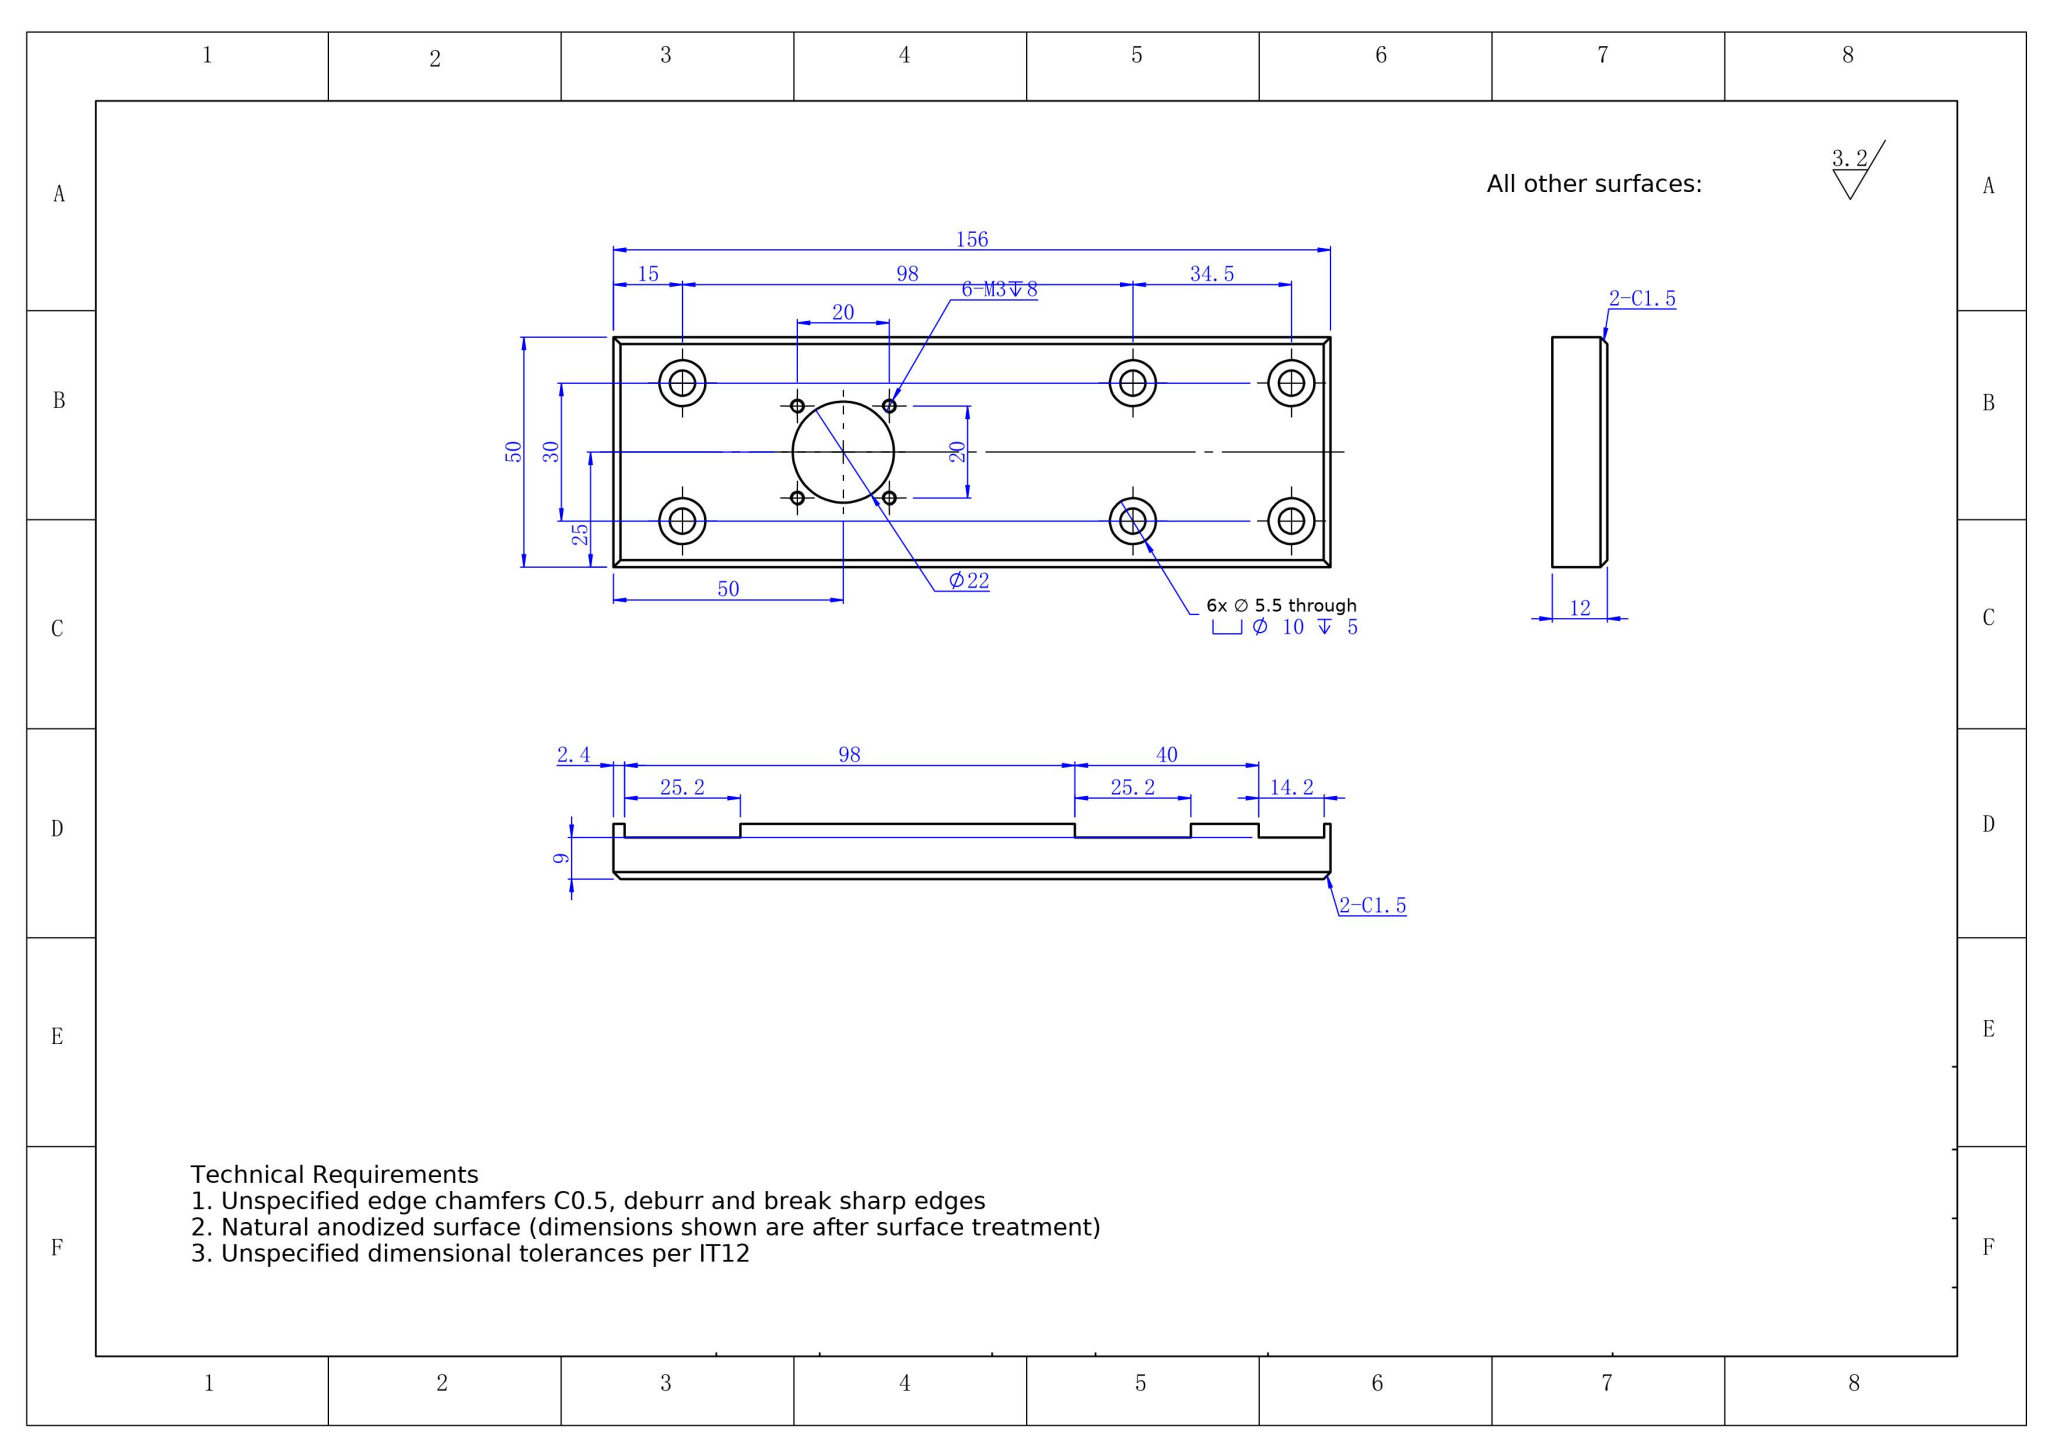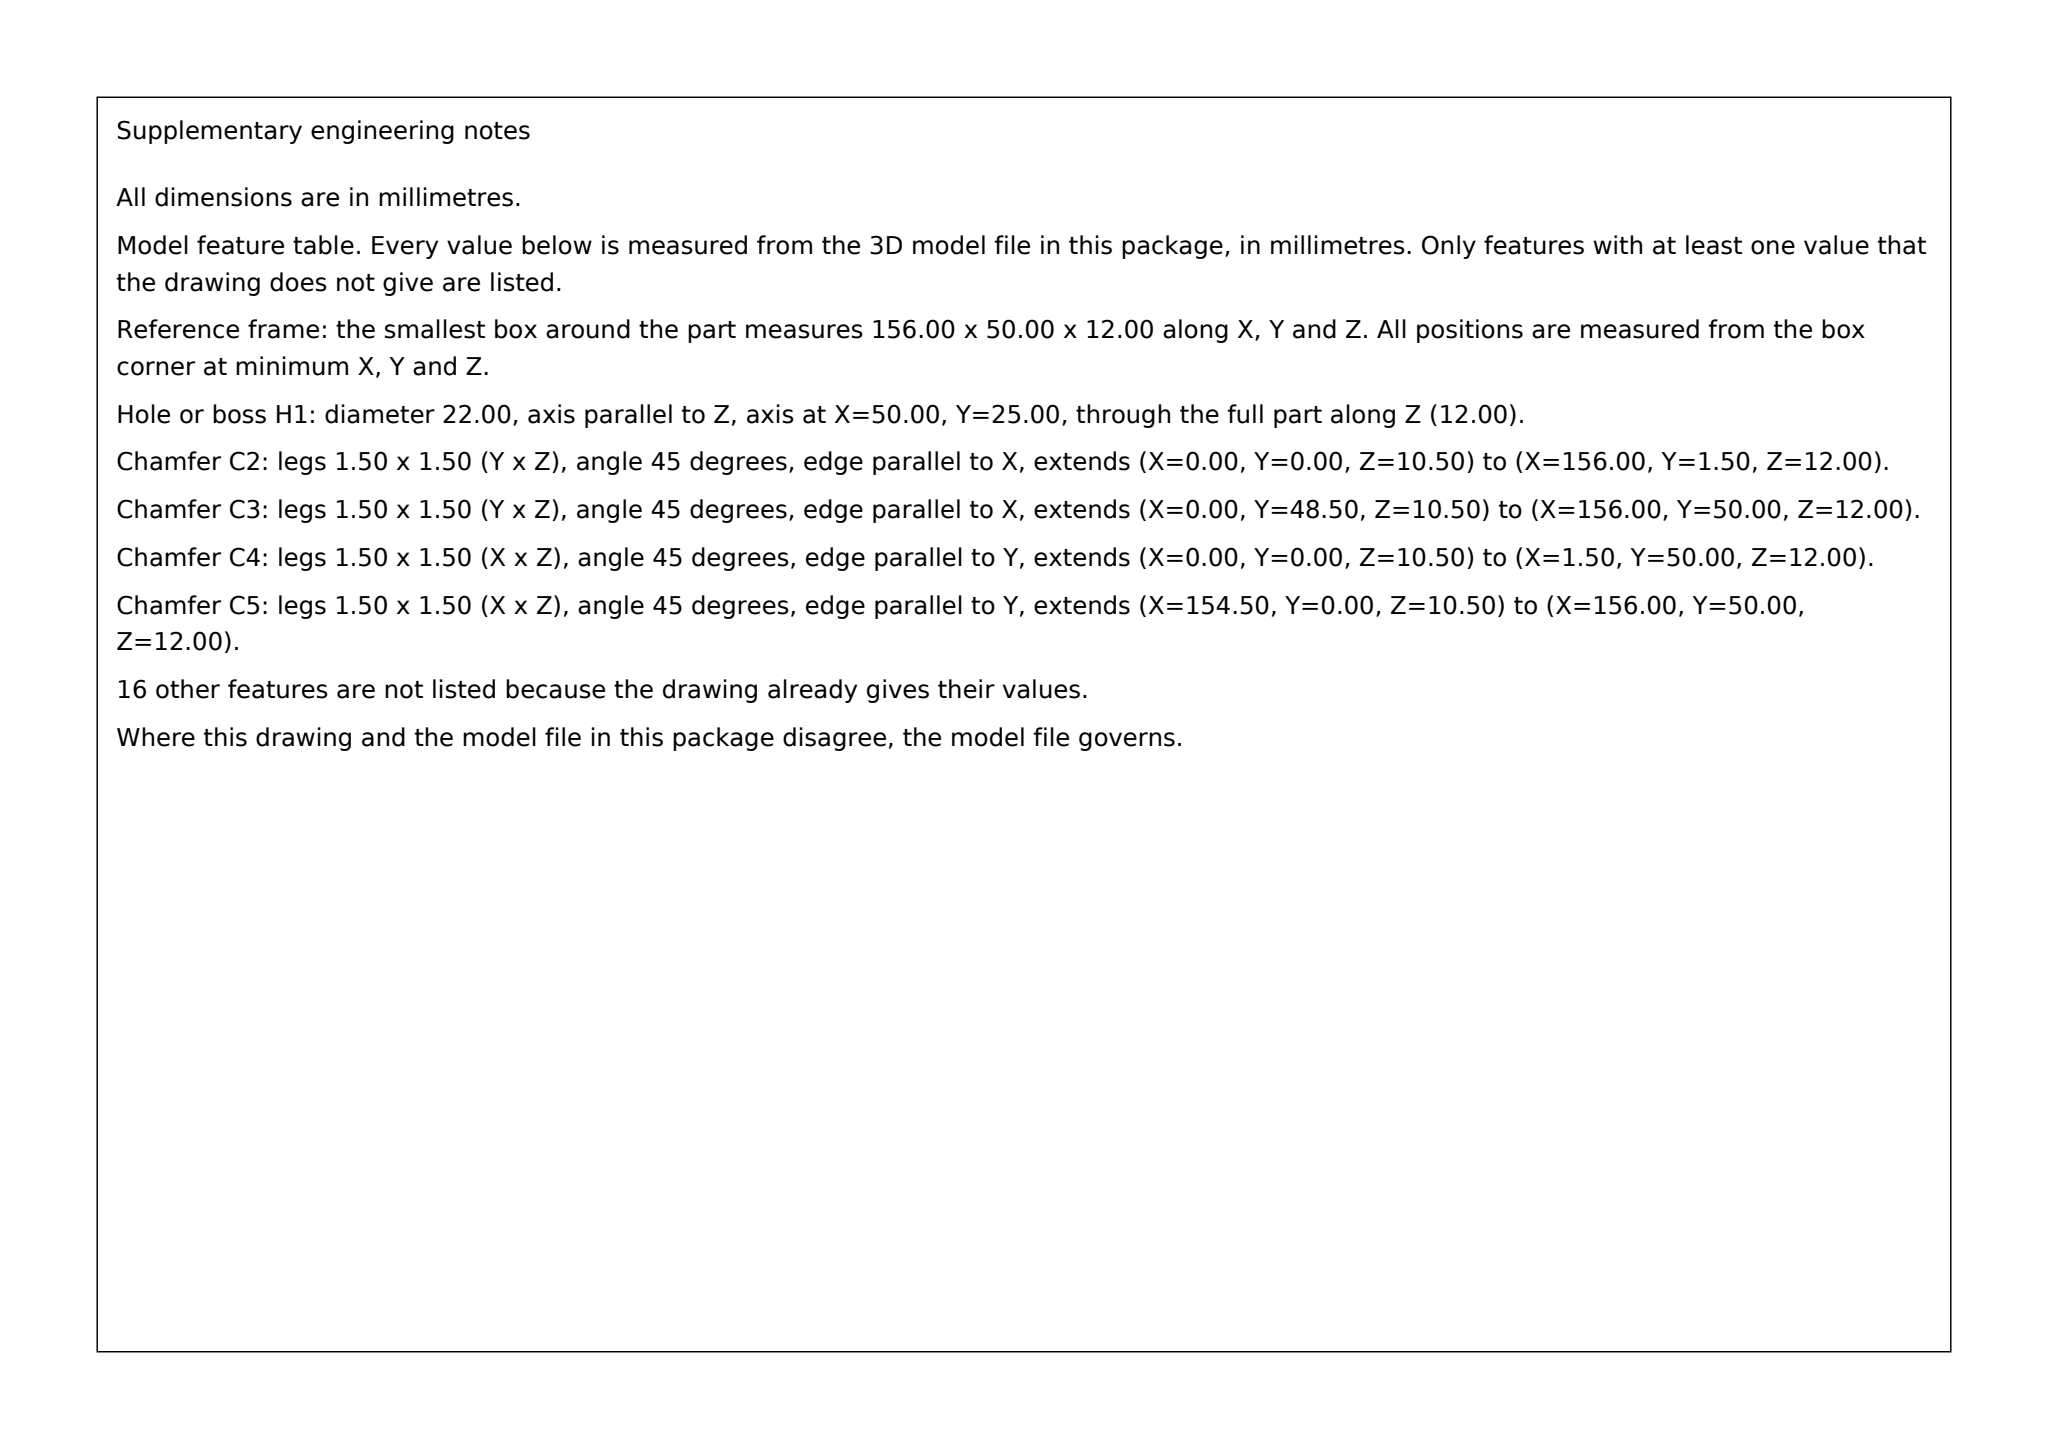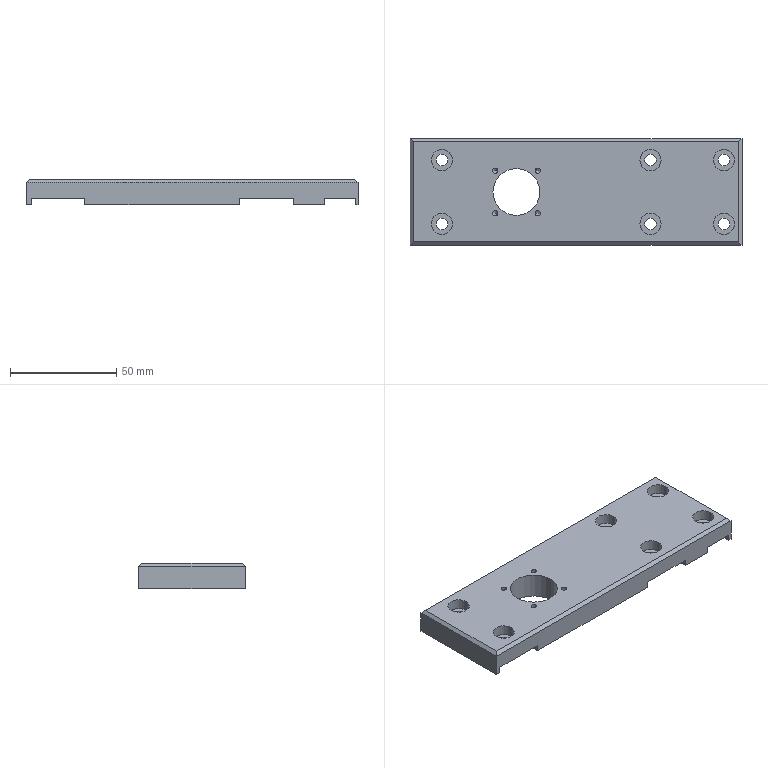Part | SolidWorks | mm | 1 solid | 70 faces | box 156 x 50 x 12 mm | volume 75811 mm3 | cylinder 34 | plane 28 | cone 8 | commonest cylinder face diameters 10 x12 5.5 x12 2.5 x8 22 x2
build123d program:
from build123d import *

# Parameters (mm, degrees)
SKETCH2_W                                  = 156
SKETCH2_H                                  = 50
BOSS_EXTRUDE2_DEPTH                        = 12
SKETCH7_W                                  = 25.2
SKETCH7_H                                  = 50
SKETCH7_W_2                                = 14.2
CUT_EXTRUDE1_DEPTH                         = 3
M5_HEX_HEAD_BOLT_COUNTERBORE_1_D           = 5.5
M5_HEX_HEAD_BOLT_COUNTERBORE_1_CBORE_D     = 10
M5_HEX_HEAD_BOLT_COUNTERBORE_1_CBORE_DEPTH = 5
SKETCH8_R                                  = 11
CUT_EXTRUDE2_DEPTH                         = 159.446
M3_TAPPED_HOLE1_D                          = 2.5
M3_TAPPED_HOLE1_DEPTH                      = 7.5
M3_TAPPED_HOLE1_TIP                        = 0.7511
CHAMFER1_SIZE                              = 1.5


with BuildPart() as part:
    # Sketch2 → Boss-Extrude2 (new body)
    with BuildSketch(Plane.XY):
        with Locations((78, 0)):
            Rectangle(SKETCH2_W, SKETCH2_H)
    extrude(amount=BOSS_EXTRUDE2_DEPTH)

    # Sketch7 → Cut-Extrude1 (cut)
    with BuildSketch(Plane(origin=(0, 0, 0), x_dir=(-1, 0, 0), z_dir=(0, 0, -1))):
        with Locations((-15, 0)):
            Rectangle(SKETCH7_W, SKETCH7_H)
        with Locations((-113, 0)):
            Rectangle(SKETCH7_W, SKETCH7_H)
        with Locations((-147.5, 0)):
            Rectangle(SKETCH7_W_2, SKETCH7_H)
    extrude(amount=-CUT_EXTRUDE1_DEPTH, mode=Mode.SUBTRACT)

    # M5 Hex Head Bolt Counterbore 1 (through all)
    with Locations(Plane.XY.offset(12)):
        with Locations((15, 15), (15, -15), (113, 15), (113, -15), (147.5, 15), (147.5, -15)):
            CounterBoreHole(M5_HEX_HEAD_BOLT_COUNTERBORE_1_D / 2, M5_HEX_HEAD_BOLT_COUNTERBORE_1_CBORE_D / 2, M5_HEX_HEAD_BOLT_COUNTERBORE_1_CBORE_DEPTH)

    # Sketch8 → Cut-Extrude2 (cut, through all)
    with BuildSketch(Plane.XY.offset(12)):
        with Locations((50, 0)):
            Circle(SKETCH8_R)
    extrude(amount=-CUT_EXTRUDE2_DEPTH, mode=Mode.SUBTRACT)

    # M3 Tapped Hole1
    with Locations(Plane.XY.offset(12)):
        with Locations((40, -10), (60, -10), (60, 10), (40, 10)):
            Hole(M3_TAPPED_HOLE1_D / 2, depth=M3_TAPPED_HOLE1_DEPTH)
            with Locations((0, 0, -(M3_TAPPED_HOLE1_DEPTH + M3_TAPPED_HOLE1_TIP / 2))):  # 118° drill point
                Cone(0, M3_TAPPED_HOLE1_D / 2, M3_TAPPED_HOLE1_TIP, mode=Mode.SUBTRACT)

    # Chamfer1
    chamfer1_edges = [part.edges().sort_by_distance(p)[0] for p in [
        (156, 0, 12),
        (78, 25, 12),
        (0, 0, 12),
        (78, -25, 12),
    ]]
    chamfer(chamfer1_edges, length=CHAMFER1_SIZE)


solid = part.part